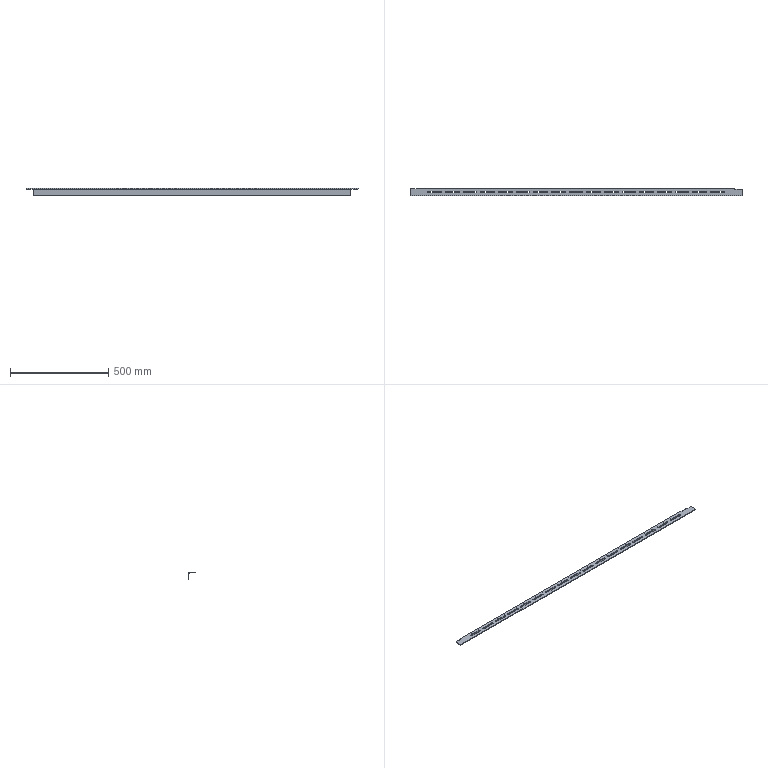Component | SolidWorks | SideFixedMountingAngleSteel-2 | 1 solid | 85 faces | box 1692 x 40 x 40 mm | volume 463911 mm3 | plane 48 | cylinder 37 | commonest cylinder face diameters 9 x34 2.667 x2 7 x1
build123d program:
from build123d import *

# Parameters (mm, degrees)
BASE_DEPTH         = 1692
SKETCH1_2_W        = 4.611
SKETCH1_2_H        = 42.038
CUT_EXTRUDE1_DEPTH = 36
SKETCH2_W          = 5.275
SKETCH2_H          = 47.654
CUT_EXTRUDE2_DEPTH = 36
CHAMFER1_SIZE      = 4
CUT_EXTRUDE3_DEPTH = 5


with BuildPart() as part:
    # Sketch1 → Base (new body)
    with BuildSketch(Plane.YZ):
        with BuildLine():
            Line((0, 40), (0, 0))
            Line((0, 0), (40, 0))
            Line((40, 0), (40, 2.667))
            ThreePointArc((40, 2.667), (39.609, 3.609), (38.667, 4))
            Line((38.667, 4), (7.5, 4))
            ThreePointArc((7.5, 4), (5.025, 5.025), (4, 7.5))
            Line((4, 7.5), (4, 38.667))
            ThreePointArc((4, 38.667), (3.609, 39.609), (2.667, 40))
            Line((2.667, 40), (0, 40))
        make_face()
    extrude(amount=BASE_DEPTH)

    # Sketch1_2 → Cut-Extrude1 (cut)
    with BuildSketch(Plane(origin=(1692, 0, 0), x_dir=(0, 0, -1), z_dir=(1, 0, 0))):
        with Locations((-2.305, 18.981)):
            Rectangle(SKETCH1_2_W, SKETCH1_2_H)
    extrude(amount=-CUT_EXTRUDE1_DEPTH, mode=Mode.SUBTRACT)

    # Sketch2 → Cut-Extrude2 (cut)
    with BuildSketch(Plane.ZY):
        with Locations((2.637, 23.827)):
            Rectangle(SKETCH2_W, SKETCH2_H)
    extrude(amount=-CUT_EXTRUDE2_DEPTH, mode=Mode.SUBTRACT)

    # Chamfer1
    chamfer1_edges = [part.edges().sort_by_distance(p)[0] for p in [
        (1692, 2.762, 4.611),
        (0, 2.399, 5.275),
    ]]
    chamfer(chamfer1_edges, length=CHAMFER1_SIZE)

    # Sketch3 → Cut-Extrude3 (cut)
    with BuildSketch(Plane.XZ):
        with BuildLine():
            Line((876.5, 15.5), (815.5, 15.5))
            ThreePointArc((815.5, 15.5), (811, 20), (815.5, 24.5))
            Line((815.5, 24.5), (876.5, 24.5))
            ThreePointArc((876.5, 24.5), (881, 20), (876.5, 15.5))
        make_face()
        with BuildLine():
            Line((966.5, 15.5), (905.5, 15.5))
            ThreePointArc((905.5, 15.5), (901, 20), (905.5, 24.5))
            Line((905.5, 24.5), (966.5, 24.5))
            ThreePointArc((966.5, 24.5), (971, 20), (966.5, 15.5))
        make_face()
        with BuildLine():
            Line((1056.5, 15.5), (995.5, 15.5))
            ThreePointArc((995.5, 15.5), (991, 20), (995.5, 24.5))
            Line((995.5, 24.5), (1056.5, 24.5))
            ThreePointArc((1056.5, 24.5), (1061, 20), (1056.5, 15.5))
        make_face()
        with BuildLine():
            Line((1146.5, 15.5), (1085.5, 15.5))
            ThreePointArc((1085.5, 15.5), (1081, 20), (1085.5, 24.5))
            Line((1085.5, 24.5), (1146.5, 24.5))
            ThreePointArc((1146.5, 24.5), (1151, 20), (1146.5, 15.5))
        make_face()
        with BuildLine():
            Line((1236.5, 15.5), (1175.5, 15.5))
            ThreePointArc((1175.5, 15.5), (1171, 20), (1175.5, 24.5))
            Line((1175.5, 24.5), (1236.5, 24.5))
            ThreePointArc((1236.5, 24.5), (1241, 20), (1236.5, 15.5))
        make_face()
        with BuildLine():
            Line((1326.5, 15.5), (1265.5, 15.5))
            ThreePointArc((1265.5, 15.5), (1261, 20), (1265.5, 24.5))
            Line((1265.5, 24.5), (1326.5, 24.5))
            ThreePointArc((1326.5, 24.5), (1331, 20), (1326.5, 15.5))
        make_face()
        with BuildLine():
            Line((1416.5, 15.5), (1355.5, 15.5))
            ThreePointArc((1355.5, 15.5), (1351, 20), (1355.5, 24.5))
            Line((1355.5, 24.5), (1416.5, 24.5))
            ThreePointArc((1416.5, 24.5), (1421, 20), (1416.5, 15.5))
        make_face()
        with BuildLine():
            Line((1506.5, 15.5), (1445.5, 15.5))
            ThreePointArc((1445.5, 15.5), (1441, 20), (1445.5, 24.5))
            Line((1445.5, 24.5), (1506.5, 24.5))
            ThreePointArc((1506.5, 24.5), (1511, 20), (1506.5, 15.5))
        make_face()
        with BuildLine():
            Line((1596.5, 15.5), (1535.5, 15.5))
            ThreePointArc((1535.5, 15.5), (1531, 20), (1535.5, 24.5))
            Line((1535.5, 24.5), (1596.5, 24.5))
            ThreePointArc((1596.5, 24.5), (1601, 20), (1596.5, 15.5))
        make_face()
        with BuildLine():
            Line((786.5, 15.5), (725.5, 15.5))
            ThreePointArc((725.5, 15.5), (721, 20), (725.5, 24.5))
            Line((725.5, 24.5), (786.5, 24.5))
            ThreePointArc((786.5, 24.5), (791, 20), (786.5, 15.5))
        make_face()
        with BuildLine():
            Line((696.5, 15.5), (635.5, 15.5))
            ThreePointArc((635.5, 15.5), (631, 20), (635.5, 24.5))
            Line((635.5, 24.5), (696.5, 24.5))
            ThreePointArc((696.5, 24.5), (701, 20), (696.5, 15.5))
        make_face()
        with BuildLine():
            Line((606.5, 15.5), (545.5, 15.5))
            ThreePointArc((545.5, 15.5), (541, 20), (545.5, 24.5))
            Line((545.5, 24.5), (606.5, 24.5))
            ThreePointArc((606.5, 24.5), (611, 20), (606.5, 15.5))
        make_face()
        with BuildLine():
            Line((516.5, 15.5), (455.5, 15.5))
            ThreePointArc((455.5, 15.5), (451, 20), (455.5, 24.5))
            Line((455.5, 24.5), (516.5, 24.5))
            ThreePointArc((516.5, 24.5), (521, 20), (516.5, 15.5))
        make_face()
        with BuildLine():
            Line((426.5, 15.5), (365.5, 15.5))
            ThreePointArc((365.5, 15.5), (361, 20), (365.5, 24.5))
            Line((365.5, 24.5), (426.5, 24.5))
            ThreePointArc((426.5, 24.5), (431, 20), (426.5, 15.5))
        make_face()
        with BuildLine():
            Line((336.5, 15.5), (275.5, 15.5))
            ThreePointArc((275.5, 15.5), (271, 20), (275.5, 24.5))
            Line((275.5, 24.5), (336.5, 24.5))
            ThreePointArc((336.5, 24.5), (341, 20), (336.5, 15.5))
        make_face()
        with BuildLine():
            Line((246.5, 15.5), (185.5, 15.5))
            ThreePointArc((185.5, 15.5), (181, 20), (185.5, 24.5))
            Line((185.5, 24.5), (246.5, 24.5))
            ThreePointArc((246.5, 24.5), (251, 20), (246.5, 15.5))
        make_face()
        with BuildLine():
            Line((156.5, 15.5), (95.5, 15.5))
            ThreePointArc((95.5, 15.5), (91, 20), (95.5, 24.5))
            Line((95.5, 24.5), (156.5, 24.5))
            ThreePointArc((156.5, 24.5), (161, 20), (156.5, 15.5))
        make_face()
    extrude(amount=-CUT_EXTRUDE3_DEPTH, mode=Mode.SUBTRACT)


solid = part.part

# Placed as in the assembly
solid = solid.moved(Location((768.152, 492.395, 98), (90, 0, -180)))